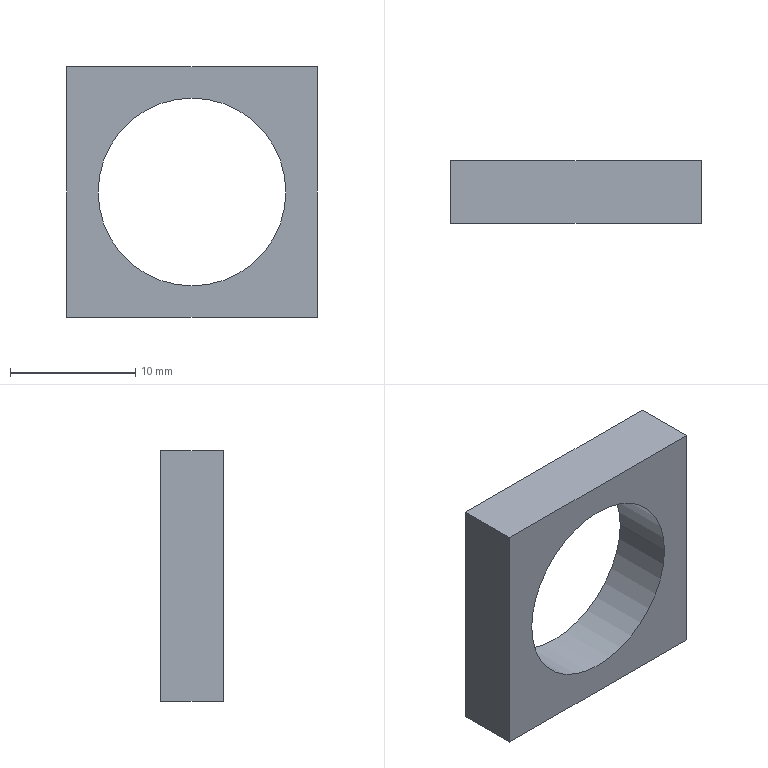Component | SolidWorks | MotorAxisHousingBase-2 | 1 solid | 8 faces | box 20 x 5 x 20 mm | volume 1116 mm3 | plane 6 | cylinder 2 | commonest cylinder face diameters 15 x2
build123d program:
from build123d import *

# Parameters (mm, degrees)
SKETCH1_W           = 20
SKETCH1_H           = 20
SKETCH1_R           = 7.5
BOSS_EXTRUDE1_DEPTH = 5


with BuildPart() as part:
    # Sketch1 → Boss-Extrude1 (new body)
    with BuildSketch(Plane.XY):
        with Locations((-263.265, -39.179)):
            Rectangle(SKETCH1_W, SKETCH1_H)
        with Locations((-263.265, -39.179)):
            Circle(SKETCH1_R, mode=Mode.SUBTRACT)
    extrude(amount=BOSS_EXTRUDE1_DEPTH)


solid = part.part

# Placed as in the assembly
solid = solid.moved(Location((528.265, 200, 69.179), (90, 0, 0)))
STEP:
#1=COLOUR_RGB('',0.7922,0.8196,0.9333);
#2=FILL_AREA_STYLE_COLOUR('',#1);
#3=FILL_AREA_STYLE('',(#2));
#4=SURFACE_STYLE_FILL_AREA(#3);
#5=SURFACE_SIDE_STYLE('',(#4));
#6=SURFACE_STYLE_USAGE(.BOTH.,#5);
#7=PRESENTATION_STYLE_ASSIGNMENT((#6));
#8=CARTESIAN_POINT('',(10.138,7.874,1.181));
#9=VERTEX_POINT('',#8);
#10=CARTESIAN_POINT('',(10.728,7.874,1.181));
#11=VERTEX_POINT('',#10);
#12=CARTESIAN_POINT('',(10.433,7.874,1.181));
#13=DIRECTION('',(0.,1.,0.));
#14=DIRECTION('',(1.,0.,0.));
#15=AXIS2_PLACEMENT_3D('',#12,#13,#14);
#16=CIRCLE('',#15,0.2953);
#17=EDGE_CURVE('',#9,#11,#16,.T.);
#18=ORIENTED_EDGE('',*,*,#17,.T.);
#19=CARTESIAN_POINT('',(10.728,7.677,1.181));
#20=VERTEX_POINT('',#19);
#21=CARTESIAN_POINT('',(10.728,7.874,1.181));
#22=DIRECTION('',(0.,-1.,0.));
#23=VECTOR('',#22,39.37);
#24=LINE('',#21,#23);
#25=EDGE_CURVE('',#11,#20,#24,.T.);
#26=ORIENTED_EDGE('',*,*,#25,.T.);
#27=CARTESIAN_POINT('',(10.138,7.677,1.181));
#28=VERTEX_POINT('',#27);
#29=CARTESIAN_POINT('',(10.433,7.677,1.181));
#30=DIRECTION('',(0.,1.,0.));
#31=DIRECTION('',(1.,0.,0.));
#32=AXIS2_PLACEMENT_3D('',#29,#30,#31);
#33=CIRCLE('',#32,0.2953);
#34=EDGE_CURVE('',#28,#20,#33,.T.);
#35=ORIENTED_EDGE('',*,*,#34,.F.);
#36=CARTESIAN_POINT('',(10.138,7.874,1.181));
#37=DIRECTION('',(0.,-1.,0.));
#38=VECTOR('',#37,39.37);
#39=LINE('',#36,#38);
#40=EDGE_CURVE('',#9,#28,#39,.T.);
#41=ORIENTED_EDGE('',*,*,#40,.F.);
#42=EDGE_LOOP('',(#18,#26,#35,#41));
#43=FACE_OUTER_BOUND('',#42,.T.);
#44=CARTESIAN_POINT('',(10.433,7.874,1.181));
#45=DIRECTION('',(0.,-1.,0.));
#46=DIRECTION('',(-1.,0.,0.));
#47=AXIS2_PLACEMENT_3D('',#44,#45,#46);
#48=CYLINDRICAL_SURFACE('',#47,0.2953);
#49=ADVANCED_FACE('',(#43),#48,.F.);
#50=CARTESIAN_POINT('',(10.827,7.874,1.575));
#51=VERTEX_POINT('',#50);
#52=CARTESIAN_POINT('',(10.827,7.874,0.7874));
#53=VERTEX_POINT('',#52);
#54=CARTESIAN_POINT('',(10.827,7.874,1.575));
#55=DIRECTION('',(0.,0.,-1.));
#56=VECTOR('',#55,39.37);
#57=LINE('',#54,#56);
#58=EDGE_CURVE('',#51,#53,#57,.T.);
#59=ORIENTED_EDGE('',*,*,#58,.T.);
#60=CARTESIAN_POINT('',(10.039,7.874,0.7874));
#61=VERTEX_POINT('',#60);
#62=CARTESIAN_POINT('',(10.039,7.874,0.7874));
#63=DIRECTION('',(-1.,0.,0.));
#64=VECTOR('',#63,39.37);
#65=LINE('',#62,#64);
#66=EDGE_CURVE('',#53,#61,#65,.T.);
#67=ORIENTED_EDGE('',*,*,#66,.T.);
#68=CARTESIAN_POINT('',(10.039,7.874,1.575));
#69=VERTEX_POINT('',#68);
#70=CARTESIAN_POINT('',(10.039,7.874,1.575));
#71=DIRECTION('',(0.,0.,1.));
#72=VECTOR('',#71,39.37);
#73=LINE('',#70,#72);
#74=EDGE_CURVE('',#61,#69,#73,.T.);
#75=ORIENTED_EDGE('',*,*,#74,.T.);
#76=CARTESIAN_POINT('',(10.039,7.874,1.575));
#77=DIRECTION('',(1.,0.,0.));
#78=VECTOR('',#77,39.37);
#79=LINE('',#76,#78);
#80=EDGE_CURVE('',#69,#51,#79,.T.);
#81=ORIENTED_EDGE('',*,*,#80,.T.);
#82=EDGE_LOOP('',(#59,#67,#75,#81));
#83=FACE_OUTER_BOUND('',#82,.T.);
#84=ORIENTED_EDGE('',*,*,#17,.F.);
#85=CARTESIAN_POINT('',(10.433,7.874,1.181));
#86=DIRECTION('',(0.,1.,0.));
#87=DIRECTION('',(1.,0.,0.));
#88=AXIS2_PLACEMENT_3D('',#85,#86,#87);
#89=CIRCLE('',#88,0.2953);
#90=EDGE_CURVE('',#11,#9,#89,.T.);
#91=ORIENTED_EDGE('',*,*,#90,.F.);
#92=EDGE_LOOP('',(#84,#91));
#93=FACE_BOUND('',#92,.T.);
#94=CARTESIAN_POINT('',(20.798,7.874,-0.3614));
#95=DIRECTION('',(0.,-1.,0.));
#96=DIRECTION('',(-1.,0.,0.));
#97=AXIS2_PLACEMENT_3D('',#94,#95,#96);
#98=PLANE('',#97);
#99=ADVANCED_FACE('',(#83,#93),#98,.F.);
#100=CARTESIAN_POINT('',(10.827,7.677,1.575));
#101=VERTEX_POINT('',#100);
#102=CARTESIAN_POINT('',(10.827,7.677,0.7874));
#103=VERTEX_POINT('',#102);
#104=CARTESIAN_POINT('',(10.827,7.677,1.575));
#105=DIRECTION('',(0.,0.,-1.));
#106=VECTOR('',#105,39.37);
#107=LINE('',#104,#106);
#108=EDGE_CURVE('',#101,#103,#107,.T.);
#109=ORIENTED_EDGE('',*,*,#108,.F.);
#110=CARTESIAN_POINT('',(10.039,7.677,1.575));
#111=VERTEX_POINT('',#110);
#112=CARTESIAN_POINT('',(10.039,7.677,1.575));
#113=DIRECTION('',(1.,0.,0.));
#114=VECTOR('',#113,39.37);
#115=LINE('',#112,#114);
#116=EDGE_CURVE('',#111,#101,#115,.T.);
#117=ORIENTED_EDGE('',*,*,#116,.F.);
#118=CARTESIAN_POINT('',(10.039,7.677,0.7874));
#119=VERTEX_POINT('',#118);
#120=CARTESIAN_POINT('',(10.039,7.677,1.575));
#121=DIRECTION('',(0.,0.,1.));
#122=VECTOR('',#121,39.37);
#123=LINE('',#120,#122);
#124=EDGE_CURVE('',#119,#111,#123,.T.);
#125=ORIENTED_EDGE('',*,*,#124,.F.);
#126=CARTESIAN_POINT('',(10.039,7.677,0.7874));
#127=DIRECTION('',(-1.,0.,0.));
#128=VECTOR('',#127,39.37);
#129=LINE('',#126,#128);
#130=EDGE_CURVE('',#103,#119,#129,.T.);
#131=ORIENTED_EDGE('',*,*,#130,.F.);
#132=EDGE_LOOP('',(#109,#117,#125,#131));
#133=FACE_OUTER_BOUND('',#132,.T.);
#134=ORIENTED_EDGE('',*,*,#34,.T.);
#135=CARTESIAN_POINT('',(10.433,7.677,1.181));
#136=DIRECTION('',(0.,1.,0.));
#137=DIRECTION('',(1.,0.,0.));
#138=AXIS2_PLACEMENT_3D('',#135,#136,#137);
#139=CIRCLE('',#138,0.2953);
#140=EDGE_CURVE('',#20,#28,#139,.T.);
#141=ORIENTED_EDGE('',*,*,#140,.T.);
#142=EDGE_LOOP('',(#134,#141));
#143=FACE_BOUND('',#142,.T.);
#144=CARTESIAN_POINT('',(20.798,7.677,-0.3614));
#145=DIRECTION('',(0.,-1.,0.));
#146=DIRECTION('',(-1.,0.,0.));
#147=AXIS2_PLACEMENT_3D('',#144,#145,#146);
#148=PLANE('',#147);
#149=ADVANCED_FACE('',(#133,#143),#148,.T.);
#150=ORIENTED_EDGE('',*,*,#108,.T.);
#151=CARTESIAN_POINT('',(10.827,7.874,0.7874));
#152=DIRECTION('',(0.,-1.,0.));
#153=VECTOR('',#152,39.37);
#154=LINE('',#151,#153);
#155=EDGE_CURVE('',#53,#103,#154,.T.);
#156=ORIENTED_EDGE('',*,*,#155,.F.);
#157=ORIENTED_EDGE('',*,*,#58,.F.);
#158=CARTESIAN_POINT('',(10.827,7.874,1.575));
#159=DIRECTION('',(0.,-1.,0.));
#160=VECTOR('',#159,39.37);
#161=LINE('',#158,#160);
#162=EDGE_CURVE('',#51,#101,#161,.T.);
#163=ORIENTED_EDGE('',*,*,#162,.T.);
#164=EDGE_LOOP('',(#150,#156,#157,#163));
#165=FACE_OUTER_BOUND('',#164,.T.);
#166=CARTESIAN_POINT('',(10.827,7.874,1.575));
#167=DIRECTION('',(-1.,0.,0.));
#168=DIRECTION('',(0.,1.,0.));
#169=AXIS2_PLACEMENT_3D('',#166,#167,#168);
#170=PLANE('',#169);
#171=ADVANCED_FACE('',(#165),#170,.F.);
#172=ORIENTED_EDGE('',*,*,#130,.T.);
#173=CARTESIAN_POINT('',(10.039,7.874,0.7874));
#174=DIRECTION('',(0.,-1.,0.));
#175=VECTOR('',#174,39.37);
#176=LINE('',#173,#175);
#177=EDGE_CURVE('',#61,#119,#176,.T.);
#178=ORIENTED_EDGE('',*,*,#177,.F.);
#179=ORIENTED_EDGE('',*,*,#66,.F.);
#180=ORIENTED_EDGE('',*,*,#155,.T.);
#181=EDGE_LOOP('',(#172,#178,#179,#180));
#182=FACE_OUTER_BOUND('',#181,.T.);
#183=CARTESIAN_POINT('',(10.039,7.874,0.7874));
#184=DIRECTION('',(0.,0.,1.));
#185=DIRECTION('',(0.,-1.,0.));
#186=AXIS2_PLACEMENT_3D('',#183,#184,#185);
#187=PLANE('',#186);
#188=ADVANCED_FACE('',(#182),#187,.F.);
#189=ORIENTED_EDGE('',*,*,#124,.T.);
#190=CARTESIAN_POINT('',(10.039,7.874,1.575));
#191=DIRECTION('',(0.,-1.,0.));
#192=VECTOR('',#191,39.37);
#193=LINE('',#190,#192);
#194=EDGE_CURVE('',#69,#111,#193,.T.);
#195=ORIENTED_EDGE('',*,*,#194,.F.);
#196=ORIENTED_EDGE('',*,*,#74,.F.);
#197=ORIENTED_EDGE('',*,*,#177,.T.);
#198=EDGE_LOOP('',(#189,#195,#196,#197));
#199=FACE_OUTER_BOUND('',#198,.T.);
#200=CARTESIAN_POINT('',(10.039,7.874,1.575));
#201=DIRECTION('',(1.,0.,0.));
#202=DIRECTION('',(0.,-1.,0.));
#203=AXIS2_PLACEMENT_3D('',#200,#201,#202);
#204=PLANE('',#203);
#205=ADVANCED_FACE('',(#199),#204,.F.);
#206=ORIENTED_EDGE('',*,*,#116,.T.);
#207=ORIENTED_EDGE('',*,*,#162,.F.);
#208=ORIENTED_EDGE('',*,*,#80,.F.);
#209=ORIENTED_EDGE('',*,*,#194,.T.);
#210=EDGE_LOOP('',(#206,#207,#208,#209));
#211=FACE_OUTER_BOUND('',#210,.T.);
#212=CARTESIAN_POINT('',(10.039,7.874,1.575));
#213=DIRECTION('',(0.,0.,-1.));
#214=DIRECTION('',(0.,1.,0.));
#215=AXIS2_PLACEMENT_3D('',#212,#213,#214);
#216=PLANE('',#215);
#217=ADVANCED_FACE('',(#211),#216,.F.);
#218=ORIENTED_EDGE('',*,*,#25,.F.);
#219=ORIENTED_EDGE('',*,*,#90,.T.);
#220=ORIENTED_EDGE('',*,*,#40,.T.);
#221=ORIENTED_EDGE('',*,*,#140,.F.);
#222=EDGE_LOOP('',(#218,#219,#220,#221));
#223=FACE_OUTER_BOUND('',#222,.T.);
#224=CARTESIAN_POINT('',(10.433,7.874,1.181));
#225=DIRECTION('',(0.,-1.,0.));
#226=DIRECTION('',(-1.,0.,0.));
#227=AXIS2_PLACEMENT_3D('',#224,#225,#226);
#228=CYLINDRICAL_SURFACE('',#227,0.2953);
#229=ADVANCED_FACE('',(#223),#228,.F.);
#230=CLOSED_SHELL('',(#49,#99,#149,#171,#188,#205,#217,#229));
#231=MANIFOLD_SOLID_BREP('',#230);
#232=STYLED_ITEM('',(#7),#231);
#233=PRESENTATION_LAYER_ASSIGNMENT('','',(#232));
#234=CARTESIAN_POINT('',(0.,0.,0.));
#235=DIRECTION('',(0.,0.,1.));
#236=DIRECTION('',(1.,0.,0.));
#237=AXIS2_PLACEMENT_3D('',#234,#235,#236);
#238=(LENGTH_UNIT()NAMED_UNIT(*)SI_UNIT($,.METRE.));
#239=LENGTH_MEASURE_WITH_UNIT(LENGTH_MEASURE(0.0254),#238);
#240=DIMENSIONAL_EXPONENTS(1.,0.,0.,0.,0.,0.,0.);
#241=(CONVERSION_BASED_UNIT('',#239)LENGTH_UNIT()NAMED_UNIT(#240));
#242=UNCERTAINTY_MEASURE_WITH_UNIT(LENGTH_MEASURE(0.00001),#241,'','');
#243=(NAMED_UNIT(*)PLANE_ANGLE_UNIT()SI_UNIT($,.RADIAN.));
#244=(NAMED_UNIT(*)SI_UNIT($,.STERADIAN.)SOLID_ANGLE_UNIT());
#245=(GEOMETRIC_REPRESENTATION_CONTEXT(3)GLOBAL_UNCERTAINTY_ASSIGNED_CONTEXT((#242))GLOBAL_UNIT_ASSIGNED_CONTEXT((#241,#243,#244))REPRESENTATION_CONTEXT('',''));
#246=ADVANCED_BREP_SHAPE_REPRESENTATION('',(#231,#237),#245);
#247=(LENGTH_UNIT()NAMED_UNIT(*)SI_UNIT($,.METRE.));
#248=LENGTH_MEASURE_WITH_UNIT(LENGTH_MEASURE(0.0254),#247);
#249=DIMENSIONAL_EXPONENTS(1.,0.,0.,0.,0.,0.,0.);
#250=(CONVERSION_BASED_UNIT('',#248)LENGTH_UNIT()NAMED_UNIT(#249));
#251=UNCERTAINTY_MEASURE_WITH_UNIT(LENGTH_MEASURE(0.00001),#250,'','');
#252=(NAMED_UNIT(*)PLANE_ANGLE_UNIT()SI_UNIT($,.RADIAN.));
#253=(NAMED_UNIT(*)SI_UNIT($,.STERADIAN.)SOLID_ANGLE_UNIT());
#254=(GEOMETRIC_REPRESENTATION_CONTEXT(3)GLOBAL_UNCERTAINTY_ASSIGNED_CONTEXT((#251))GLOBAL_UNIT_ASSIGNED_CONTEXT((#250,#252,#253))REPRESENTATION_CONTEXT('',''));
#255=MECHANICAL_DESIGN_GEOMETRIC_PRESENTATION_REPRESENTATION('',(#232),#254);